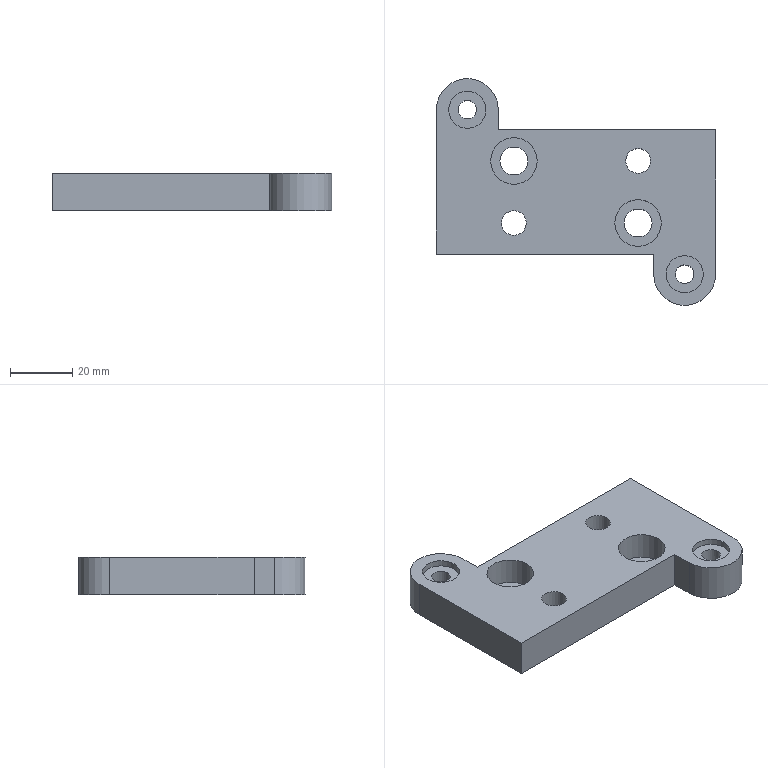Component | NX | DATUM_BLOCK | 1 solid | 24 faces | volume 44348 mm3 | cylinder 12 | plane 12 | commonest cylinder face diameters 6 x2 20 x2 12 x2 9 x2 15 x2 8 x2